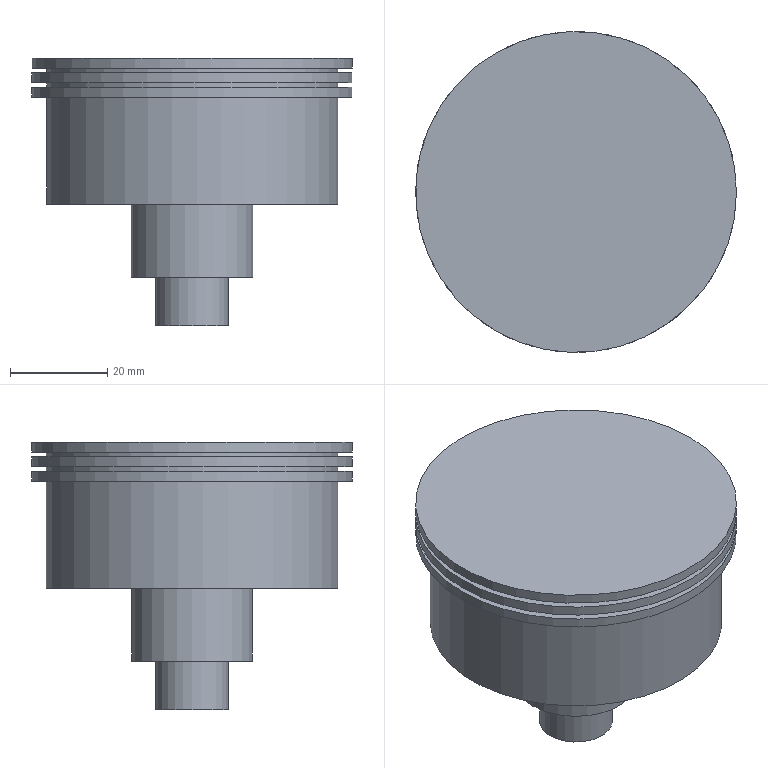Component | NX | AIR_PUMP | 1 solid | 17 faces | box 66 x 66 x 55 mm | volume 97516 mm3 | plane 9 | cylinder 8 | commonest cylinder face diameters 66 x3 60 x3 25 x1 15 x1
STEP:
#1=CARTESIAN_POINT('',(0.,0.,0.));
#2=DIRECTION('',(0.,0.,1.));
#3=DIRECTION('',(1.,0.,0.));
#4=AXIS2_PLACEMENT_3D('',#1,#2,#3);
#5=CARTESIAN_POINT('',(73.907,-56.768,202.5));
#6=VERTEX_POINT('',#5);
#7=CARTESIAN_POINT('',(70.,-24.,202.5));
#8=DIRECTION('',(0.,0.,-1.));
#9=DIRECTION('',(0.1184,-0.993,0.));
#10=AXIS2_PLACEMENT_3D('',#7,#8,#9);
#11=CIRCLE('',#10,33.);
#12=CARTESIAN_POINT('',(70.,-24.,202.5));
#13=DIRECTION('',(0.,0.,1.));
#14=DIRECTION('',(0.1184,-0.993,0.));
#15=AXIS2_PLACEMENT_3D('',#12,#13,#14);
#16=PLANE('',#15);
#17=CARTESIAN_POINT('',(33.,0.));
#18=CARTESIAN_POINT('',(33.,-57.158));
#19=CARTESIAN_POINT('',(-16.5,-28.579));
#20=CARTESIAN_POINT('',(-66.,-0.));
#21=CARTESIAN_POINT('',(-16.5,28.579));
#22=CARTESIAN_POINT('',(33.,57.158));
#23=CARTESIAN_POINT('',(33.,0.));
#24=(BOUNDED_CURVE()B_SPLINE_CURVE(2,(#17,#18,#19,#20,#21,#22,#23),.UNSPECIFIED.,.T.,.F.)B_SPLINE_CURVE_WITH_KNOTS((1,2,2,2,2,1),(-2.094,0.,2.094,4.189,6.283,8.378),.UNSPECIFIED.)CURVE()GEOMETRIC_REPRESENTATION_ITEM()RATIONAL_B_SPLINE_CURVE((1.,0.5,1.,0.5,1.,0.5,1.))REPRESENTATION_ITEM(''));
#25=(GEOMETRIC_REPRESENTATION_CONTEXT(2)PARAMETRIC_REPRESENTATION_CONTEXT()REPRESENTATION_CONTEXT('',''));
#26=DEFINITIONAL_REPRESENTATION('',(#24),#25);
#27=PCURVE('',#16,#26);
#28=CARTESIAN_POINT('',(70.,-24.,200.5));
#29=DIRECTION('',(0.,0.,1.));
#30=DIRECTION('',(0.1184,-0.993,0.));
#31=AXIS2_PLACEMENT_3D('',#28,#29,#30);
#32=CYLINDRICAL_SURFACE('',#31,33.);
#33=CARTESIAN_POINT('',(6.283,2.));
#34=DIRECTION('',(-1.,0.));
#35=VECTOR('',#34,1.);
#36=LINE('',#33,#35);
#37=(GEOMETRIC_REPRESENTATION_CONTEXT(2)PARAMETRIC_REPRESENTATION_CONTEXT()REPRESENTATION_CONTEXT('',''));
#38=DEFINITIONAL_REPRESENTATION('',(#36),#37);
#39=PCURVE('',#32,#38);
#40=SURFACE_CURVE('',#11,(#27,#39),.PCURVE_S1.);
#41=EDGE_CURVE('',#6,#6,#40,.T.);
#42=ORIENTED_EDGE('',*,*,#41,.F.);
#43=EDGE_LOOP('',(#42));
#44=FACE_BOUND('',#43,.T.);
#45=ADVANCED_FACE('',(#44),#16,.T.);
#46=CARTESIAN_POINT('',(66.448,5.789,200.5));
#47=VERTEX_POINT('',#46);
#48=CARTESIAN_POINT('',(70.,-24.,200.5));
#49=DIRECTION('',(0.,0.,-1.));
#50=DIRECTION('',(-0.1184,0.993,0.));
#51=AXIS2_PLACEMENT_3D('',#48,#49,#50);
#52=CIRCLE('',#51,30.);
#53=CARTESIAN_POINT('',(70.,-24.,200.5));
#54=DIRECTION('',(0.,0.,-1.));
#55=DIRECTION('',(-0.1184,0.993,0.));
#56=AXIS2_PLACEMENT_3D('',#53,#54,#55);
#57=PLANE('',#56);
#58=CARTESIAN_POINT('',(0.,0.));
#59=DIRECTION('',(1.,0.));
#60=AXIS2_PLACEMENT_2D('',#58,#59);
#61=CIRCLE('',#60,30.);
#62=(GEOMETRIC_REPRESENTATION_CONTEXT(2)PARAMETRIC_REPRESENTATION_CONTEXT()REPRESENTATION_CONTEXT('',''));
#63=DEFINITIONAL_REPRESENTATION('',(#61),#62);
#64=PCURVE('',#57,#63);
#65=CARTESIAN_POINT('',(70.,-24.,200.5));
#66=DIRECTION('',(0.,0.,-1.));
#67=DIRECTION('',(-0.1184,0.993,0.));
#68=AXIS2_PLACEMENT_3D('',#65,#66,#67);
#69=CYLINDRICAL_SURFACE('',#68,30.);
#70=CARTESIAN_POINT('',(0.,0.));
#71=DIRECTION('',(1.,0.));
#72=VECTOR('',#71,1.);
#73=LINE('',#70,#72);
#74=(GEOMETRIC_REPRESENTATION_CONTEXT(2)PARAMETRIC_REPRESENTATION_CONTEXT()REPRESENTATION_CONTEXT('',''));
#75=DEFINITIONAL_REPRESENTATION('',(#73),#74);
#76=PCURVE('',#69,#75);
#77=SURFACE_CURVE('',#52,(#64,#76),.PCURVE_S1.);
#78=EDGE_CURVE('',#47,#47,#77,.T.);
#79=ORIENTED_EDGE('',*,*,#78,.F.);
#80=EDGE_LOOP('',(#79));
#81=FACE_BOUND('',#80,.T.);
#82=CARTESIAN_POINT('',(73.907,-56.768,200.5));
#83=VERTEX_POINT('',#82);
#84=CARTESIAN_POINT('',(70.,-24.,200.5));
#85=DIRECTION('',(0.,0.,1.));
#86=DIRECTION('',(0.1184,-0.993,0.));
#87=AXIS2_PLACEMENT_3D('',#84,#85,#86);
#88=CIRCLE('',#87,33.);
#89=CARTESIAN_POINT('',(-33.,0.));
#90=CARTESIAN_POINT('',(-33.,57.158));
#91=CARTESIAN_POINT('',(16.5,28.579));
#92=CARTESIAN_POINT('',(66.,0.));
#93=CARTESIAN_POINT('',(16.5,-28.579));
#94=CARTESIAN_POINT('',(-33.,-57.158));
#95=CARTESIAN_POINT('',(-33.,0.));
#96=(BOUNDED_CURVE()B_SPLINE_CURVE(2,(#89,#90,#91,#92,#93,#94,#95),.UNSPECIFIED.,.T.,.F.)B_SPLINE_CURVE_WITH_KNOTS((1,2,2,2,2,1),(-2.094,0.,2.094,4.189,6.283,8.378),.UNSPECIFIED.)CURVE()GEOMETRIC_REPRESENTATION_ITEM()RATIONAL_B_SPLINE_CURVE((1.,0.5,1.,0.5,1.,0.5,1.))REPRESENTATION_ITEM(''));
#97=(GEOMETRIC_REPRESENTATION_CONTEXT(2)PARAMETRIC_REPRESENTATION_CONTEXT()REPRESENTATION_CONTEXT('',''));
#98=DEFINITIONAL_REPRESENTATION('',(#96),#97);
#99=PCURVE('',#57,#98);
#100=CARTESIAN_POINT('',(0.,0.));
#101=DIRECTION('',(1.,0.));
#102=VECTOR('',#101,1.);
#103=LINE('',#100,#102);
#104=(GEOMETRIC_REPRESENTATION_CONTEXT(2)PARAMETRIC_REPRESENTATION_CONTEXT()REPRESENTATION_CONTEXT('',''));
#105=DEFINITIONAL_REPRESENTATION('',(#103),#104);
#106=PCURVE('',#32,#105);
#107=SURFACE_CURVE('',#88,(#99,#106),.PCURVE_S1.);
#108=EDGE_CURVE('',#83,#83,#107,.T.);
#109=ORIENTED_EDGE('',*,*,#108,.F.);
#110=EDGE_LOOP('',(#109));
#111=FACE_BOUND('',#110,.T.);
#112=ADVANCED_FACE('',(#81,#111),#57,.T.);
#113=ORIENTED_EDGE('',*,*,#41,.T.);
#114=CARTESIAN_POINT('',(73.907,-56.768,200.5));
#115=CARTESIAN_POINT('',(73.907,-56.768,202.5));
#116=B_SPLINE_CURVE_WITH_KNOTS('',1,(#114,#115),.UNSPECIFIED.,.F.,.F.,(2,2),(0.,2.),.PIECEWISE_BEZIER_KNOTS.);
#117=CARTESIAN_POINT('',(0.,0.));
#118=DIRECTION('',(0.,1.));
#119=VECTOR('',#118,1.);
#120=LINE('',#117,#119);
#121=(GEOMETRIC_REPRESENTATION_CONTEXT(2)PARAMETRIC_REPRESENTATION_CONTEXT()REPRESENTATION_CONTEXT('',''));
#122=DEFINITIONAL_REPRESENTATION('',(#120),#121);
#123=PCURVE('',#32,#122);
#124=CARTESIAN_POINT('',(6.283,0.));
#125=DIRECTION('',(0.,1.));
#126=VECTOR('',#125,1.);
#127=LINE('',#124,#126);
#128=(GEOMETRIC_REPRESENTATION_CONTEXT(2)PARAMETRIC_REPRESENTATION_CONTEXT()REPRESENTATION_CONTEXT('',''));
#129=DEFINITIONAL_REPRESENTATION('',(#127),#128);
#130=PCURVE('',#32,#129);
#131=SEAM_CURVE('',#116,(#123,#130),.PCURVE_S1.);
#132=EDGE_CURVE('',#83,#6,#131,.T.);
#133=ORIENTED_EDGE('',*,*,#132,.F.);
#134=ORIENTED_EDGE('',*,*,#108,.T.);
#135=ORIENTED_EDGE('',*,*,#132,.T.);
#136=EDGE_LOOP('',(#113,#133,#134,#135));
#137=FACE_BOUND('',#136,.T.);
#138=ADVANCED_FACE('',(#137),#32,.T.);
#139=CARTESIAN_POINT('',(66.448,5.789,199.5));
#140=VERTEX_POINT('',#139);
#141=CARTESIAN_POINT('',(70.,-24.,199.5));
#142=DIRECTION('',(0.,0.,-1.));
#143=DIRECTION('',(-0.1184,0.993,0.));
#144=AXIS2_PLACEMENT_3D('',#141,#142,#143);
#145=CIRCLE('',#144,30.);
#146=CARTESIAN_POINT('',(0.,1.));
#147=DIRECTION('',(1.,0.));
#148=VECTOR('',#147,1.);
#149=LINE('',#146,#148);
#150=(GEOMETRIC_REPRESENTATION_CONTEXT(2)PARAMETRIC_REPRESENTATION_CONTEXT()REPRESENTATION_CONTEXT('',''));
#151=DEFINITIONAL_REPRESENTATION('',(#149),#150);
#152=PCURVE('',#69,#151);
#153=CARTESIAN_POINT('',(70.,-24.,199.5));
#154=DIRECTION('',(0.,0.,1.));
#155=DIRECTION('',(0.1184,-0.993,0.));
#156=AXIS2_PLACEMENT_3D('',#153,#154,#155);
#157=PLANE('',#156);
#158=CARTESIAN_POINT('',(-30.,0.));
#159=CARTESIAN_POINT('',(-30.,51.962));
#160=CARTESIAN_POINT('',(15.,25.981));
#161=CARTESIAN_POINT('',(60.,0.));
#162=CARTESIAN_POINT('',(15.,-25.981));
#163=CARTESIAN_POINT('',(-30.,-51.962));
#164=CARTESIAN_POINT('',(-30.,0.));
#165=(BOUNDED_CURVE()B_SPLINE_CURVE(2,(#158,#159,#160,#161,#162,#163,#164),.UNSPECIFIED.,.T.,.F.)B_SPLINE_CURVE_WITH_KNOTS((1,2,2,2,2,1),(-2.094,0.,2.094,4.189,6.283,8.378),.UNSPECIFIED.)CURVE()GEOMETRIC_REPRESENTATION_ITEM()RATIONAL_B_SPLINE_CURVE((1.,0.5,1.,0.5,1.,0.5,1.))REPRESENTATION_ITEM(''));
#166=(GEOMETRIC_REPRESENTATION_CONTEXT(2)PARAMETRIC_REPRESENTATION_CONTEXT()REPRESENTATION_CONTEXT('',''));
#167=DEFINITIONAL_REPRESENTATION('',(#165),#166);
#168=PCURVE('',#157,#167);
#169=SURFACE_CURVE('',#145,(#152,#168),.PCURVE_S1.);
#170=EDGE_CURVE('',#140,#140,#169,.T.);
#171=ORIENTED_EDGE('',*,*,#170,.F.);
#172=CARTESIAN_POINT('',(66.448,5.789,200.5));
#173=CARTESIAN_POINT('',(66.448,5.789,199.5));
#174=B_SPLINE_CURVE_WITH_KNOTS('',1,(#172,#173),.UNSPECIFIED.,.F.,.F.,(2,2),(0.,1.),.PIECEWISE_BEZIER_KNOTS.);
#175=CARTESIAN_POINT('',(0.,0.));
#176=DIRECTION('',(0.,1.));
#177=VECTOR('',#176,1.);
#178=LINE('',#175,#177);
#179=(GEOMETRIC_REPRESENTATION_CONTEXT(2)PARAMETRIC_REPRESENTATION_CONTEXT()REPRESENTATION_CONTEXT('',''));
#180=DEFINITIONAL_REPRESENTATION('',(#178),#179);
#181=PCURVE('',#69,#180);
#182=CARTESIAN_POINT('',(6.283,0.));
#183=DIRECTION('',(0.,1.));
#184=VECTOR('',#183,1.);
#185=LINE('',#182,#184);
#186=(GEOMETRIC_REPRESENTATION_CONTEXT(2)PARAMETRIC_REPRESENTATION_CONTEXT()REPRESENTATION_CONTEXT('',''));
#187=DEFINITIONAL_REPRESENTATION('',(#185),#186);
#188=PCURVE('',#69,#187);
#189=SEAM_CURVE('',#174,(#181,#188),.PCURVE_S1.);
#190=EDGE_CURVE('',#47,#140,#189,.T.);
#191=ORIENTED_EDGE('',*,*,#190,.F.);
#192=ORIENTED_EDGE('',*,*,#78,.T.);
#193=ORIENTED_EDGE('',*,*,#190,.T.);
#194=EDGE_LOOP('',(#171,#191,#192,#193));
#195=FACE_BOUND('',#194,.T.);
#196=ADVANCED_FACE('',(#195),#69,.T.);
#197=CARTESIAN_POINT('',(66.448,5.789,197.5));
#198=VERTEX_POINT('',#197);
#199=CARTESIAN_POINT('',(70.,-24.,197.5));
#200=DIRECTION('',(0.,0.,-1.));
#201=DIRECTION('',(-0.1184,0.993,0.));
#202=AXIS2_PLACEMENT_3D('',#199,#200,#201);
#203=CIRCLE('',#202,30.);
#204=CARTESIAN_POINT('',(70.,-24.,197.5));
#205=DIRECTION('',(0.,0.,-1.));
#206=DIRECTION('',(-0.1184,0.993,0.));
#207=AXIS2_PLACEMENT_3D('',#204,#205,#206);
#208=PLANE('',#207);
#209=CARTESIAN_POINT('',(0.,0.));
#210=DIRECTION('',(1.,0.));
#211=AXIS2_PLACEMENT_2D('',#209,#210);
#212=CIRCLE('',#211,30.);
#213=(GEOMETRIC_REPRESENTATION_CONTEXT(2)PARAMETRIC_REPRESENTATION_CONTEXT()REPRESENTATION_CONTEXT('',''));
#214=DEFINITIONAL_REPRESENTATION('',(#212),#213);
#215=PCURVE('',#208,#214);
#216=CARTESIAN_POINT('',(70.,-24.,197.5));
#217=DIRECTION('',(0.,0.,-1.));
#218=DIRECTION('',(-0.1184,0.993,0.));
#219=AXIS2_PLACEMENT_3D('',#216,#217,#218);
#220=CYLINDRICAL_SURFACE('',#219,30.);
#221=CARTESIAN_POINT('',(0.,0.));
#222=DIRECTION('',(1.,0.));
#223=VECTOR('',#222,1.);
#224=LINE('',#221,#223);
#225=(GEOMETRIC_REPRESENTATION_CONTEXT(2)PARAMETRIC_REPRESENTATION_CONTEXT()REPRESENTATION_CONTEXT('',''));
#226=DEFINITIONAL_REPRESENTATION('',(#224),#225);
#227=PCURVE('',#220,#226);
#228=SURFACE_CURVE('',#203,(#215,#227),.PCURVE_S1.);
#229=EDGE_CURVE('',#198,#198,#228,.T.);
#230=ORIENTED_EDGE('',*,*,#229,.F.);
#231=EDGE_LOOP('',(#230));
#232=FACE_BOUND('',#231,.T.);
#233=CARTESIAN_POINT('',(66.093,8.768,197.5));
#234=VERTEX_POINT('',#233);
#235=CARTESIAN_POINT('',(70.,-24.,197.5));
#236=DIRECTION('',(0.,0.,-1.));
#237=DIRECTION('',(-0.1184,0.993,0.));
#238=AXIS2_PLACEMENT_3D('',#235,#236,#237);
#239=CIRCLE('',#238,33.);
#240=CARTESIAN_POINT('',(0.,0.));
#241=DIRECTION('',(1.,0.));
#242=AXIS2_PLACEMENT_2D('',#240,#241);
#243=CIRCLE('',#242,33.);
#244=(GEOMETRIC_REPRESENTATION_CONTEXT(2)PARAMETRIC_REPRESENTATION_CONTEXT()REPRESENTATION_CONTEXT('',''));
#245=DEFINITIONAL_REPRESENTATION('',(#243),#244);
#246=PCURVE('',#208,#245);
#247=CARTESIAN_POINT('',(70.,-24.,199.5));
#248=DIRECTION('',(0.,0.,-1.));
#249=DIRECTION('',(-0.1184,0.993,0.));
#250=AXIS2_PLACEMENT_3D('',#247,#248,#249);
#251=CYLINDRICAL_SURFACE('',#250,33.);
#252=CARTESIAN_POINT('',(0.,2.));
#253=DIRECTION('',(1.,0.));
#254=VECTOR('',#253,1.);
#255=LINE('',#252,#254);
#256=(GEOMETRIC_REPRESENTATION_CONTEXT(2)PARAMETRIC_REPRESENTATION_CONTEXT()REPRESENTATION_CONTEXT('',''));
#257=DEFINITIONAL_REPRESENTATION('',(#255),#256);
#258=PCURVE('',#251,#257);
#259=SURFACE_CURVE('',#239,(#246,#258),.PCURVE_S1.);
#260=EDGE_CURVE('',#234,#234,#259,.T.);
#261=ORIENTED_EDGE('',*,*,#260,.T.);
#262=EDGE_LOOP('',(#261));
#263=FACE_BOUND('',#262,.T.);
#264=ADVANCED_FACE('',(#232,#263),#208,.T.);
#265=ORIENTED_EDGE('',*,*,#170,.T.);
#266=EDGE_LOOP('',(#265));
#267=FACE_BOUND('',#266,.T.);
#268=CARTESIAN_POINT('',(66.093,8.768,199.5));
#269=VERTEX_POINT('',#268);
#270=CARTESIAN_POINT('',(70.,-24.,199.5));
#271=DIRECTION('',(0.,0.,-1.));
#272=DIRECTION('',(-0.1184,0.993,0.));
#273=AXIS2_PLACEMENT_3D('',#270,#271,#272);
#274=CIRCLE('',#273,33.);
#275=CARTESIAN_POINT('',(-33.,0.));
#276=CARTESIAN_POINT('',(-33.,57.158));
#277=CARTESIAN_POINT('',(16.5,28.579));
#278=CARTESIAN_POINT('',(66.,0.));
#279=CARTESIAN_POINT('',(16.5,-28.579));
#280=CARTESIAN_POINT('',(-33.,-57.158));
#281=CARTESIAN_POINT('',(-33.,0.));
#282=(BOUNDED_CURVE()B_SPLINE_CURVE(2,(#275,#276,#277,#278,#279,#280,#281),.UNSPECIFIED.,.T.,.F.)B_SPLINE_CURVE_WITH_KNOTS((1,2,2,2,2,1),(-2.094,0.,2.094,4.189,6.283,8.378),.UNSPECIFIED.)CURVE()GEOMETRIC_REPRESENTATION_ITEM()RATIONAL_B_SPLINE_CURVE((1.,0.5,1.,0.5,1.,0.5,1.))REPRESENTATION_ITEM(''));
#283=(GEOMETRIC_REPRESENTATION_CONTEXT(2)PARAMETRIC_REPRESENTATION_CONTEXT()REPRESENTATION_CONTEXT('',''));
#284=DEFINITIONAL_REPRESENTATION('',(#282),#283);
#285=PCURVE('',#157,#284);
#286=CARTESIAN_POINT('',(0.,0.));
#287=DIRECTION('',(1.,0.));
#288=VECTOR('',#287,1.);
#289=LINE('',#286,#288);
#290=(GEOMETRIC_REPRESENTATION_CONTEXT(2)PARAMETRIC_REPRESENTATION_CONTEXT()REPRESENTATION_CONTEXT('',''));
#291=DEFINITIONAL_REPRESENTATION('',(#289),#290);
#292=PCURVE('',#251,#291);
#293=SURFACE_CURVE('',#274,(#285,#292),.PCURVE_S1.);
#294=EDGE_CURVE('',#269,#269,#293,.T.);
#295=ORIENTED_EDGE('',*,*,#294,.F.);
#296=EDGE_LOOP('',(#295));
#297=FACE_BOUND('',#296,.T.);
#298=ADVANCED_FACE('',(#267,#297),#157,.T.);
#299=ORIENTED_EDGE('',*,*,#260,.F.);
#300=CARTESIAN_POINT('',(66.093,8.768,199.5));
#301=CARTESIAN_POINT('',(66.093,8.768,197.5));
#302=B_SPLINE_CURVE_WITH_KNOTS('',1,(#300,#301),.UNSPECIFIED.,.F.,.F.,(2,2),(0.,2.),.PIECEWISE_BEZIER_KNOTS.);
#303=CARTESIAN_POINT('',(0.,0.));
#304=DIRECTION('',(0.,1.));
#305=VECTOR('',#304,1.);
#306=LINE('',#303,#305);
#307=(GEOMETRIC_REPRESENTATION_CONTEXT(2)PARAMETRIC_REPRESENTATION_CONTEXT()REPRESENTATION_CONTEXT('',''));
#308=DEFINITIONAL_REPRESENTATION('',(#306),#307);
#309=PCURVE('',#251,#308);
#310=CARTESIAN_POINT('',(6.283,0.));
#311=DIRECTION('',(0.,1.));
#312=VECTOR('',#311,1.);
#313=LINE('',#310,#312);
#314=(GEOMETRIC_REPRESENTATION_CONTEXT(2)PARAMETRIC_REPRESENTATION_CONTEXT()REPRESENTATION_CONTEXT('',''));
#315=DEFINITIONAL_REPRESENTATION('',(#313),#314);
#316=PCURVE('',#251,#315);
#317=SEAM_CURVE('',#302,(#309,#316),.PCURVE_S1.);
#318=EDGE_CURVE('',#269,#234,#317,.T.);
#319=ORIENTED_EDGE('',*,*,#318,.F.);
#320=ORIENTED_EDGE('',*,*,#294,.T.);
#321=ORIENTED_EDGE('',*,*,#318,.T.);
#322=EDGE_LOOP('',(#299,#319,#320,#321));
#323=FACE_BOUND('',#322,.T.);
#324=ADVANCED_FACE('',(#323),#251,.T.);
#325=CARTESIAN_POINT('',(66.448,5.789,196.5));
#326=VERTEX_POINT('',#325);
#327=CARTESIAN_POINT('',(70.,-24.,196.5));
#328=DIRECTION('',(0.,0.,-1.));
#329=DIRECTION('',(-0.1184,0.993,0.));
#330=AXIS2_PLACEMENT_3D('',#327,#328,#329);
#331=CIRCLE('',#330,30.);
#332=CARTESIAN_POINT('',(0.,1.));
#333=DIRECTION('',(1.,0.));
#334=VECTOR('',#333,1.);
#335=LINE('',#332,#334);
#336=(GEOMETRIC_REPRESENTATION_CONTEXT(2)PARAMETRIC_REPRESENTATION_CONTEXT()REPRESENTATION_CONTEXT('',''));
#337=DEFINITIONAL_REPRESENTATION('',(#335),#336);
#338=PCURVE('',#220,#337);
#339=CARTESIAN_POINT('',(70.,-24.,196.5));
#340=DIRECTION('',(0.,0.,1.));
#341=DIRECTION('',(0.1184,-0.993,0.));
#342=AXIS2_PLACEMENT_3D('',#339,#340,#341);
#343=PLANE('',#342);
#344=CARTESIAN_POINT('',(-30.,0.));
#345=CARTESIAN_POINT('',(-30.,51.962));
#346=CARTESIAN_POINT('',(15.,25.981));
#347=CARTESIAN_POINT('',(60.,0.));
#348=CARTESIAN_POINT('',(15.,-25.981));
#349=CARTESIAN_POINT('',(-30.,-51.962));
#350=CARTESIAN_POINT('',(-30.,0.));
#351=(BOUNDED_CURVE()B_SPLINE_CURVE(2,(#344,#345,#346,#347,#348,#349,#350),.UNSPECIFIED.,.T.,.F.)B_SPLINE_CURVE_WITH_KNOTS((1,2,2,2,2,1),(-2.094,0.,2.094,4.189,6.283,8.378),.UNSPECIFIED.)CURVE()GEOMETRIC_REPRESENTATION_ITEM()RATIONAL_B_SPLINE_CURVE((1.,0.5,1.,0.5,1.,0.5,1.))REPRESENTATION_ITEM(''));
#352=(GEOMETRIC_REPRESENTATION_CONTEXT(2)PARAMETRIC_REPRESENTATION_CONTEXT()REPRESENTATION_CONTEXT('',''));
#353=DEFINITIONAL_REPRESENTATION('',(#351),#352);
#354=PCURVE('',#343,#353);
#355=SURFACE_CURVE('',#331,(#338,#354),.PCURVE_S1.);
#356=EDGE_CURVE('',#326,#326,#355,.T.);
#357=ORIENTED_EDGE('',*,*,#356,.F.);
#358=CARTESIAN_POINT('',(66.448,5.789,197.5));
#359=CARTESIAN_POINT('',(66.448,5.789,196.5));
#360=B_SPLINE_CURVE_WITH_KNOTS('',1,(#358,#359),.UNSPECIFIED.,.F.,.F.,(2,2),(0.,1.),.PIECEWISE_BEZIER_KNOTS.);
#361=CARTESIAN_POINT('',(0.,0.));
#362=DIRECTION('',(0.,1.));
#363=VECTOR('',#362,1.);
#364=LINE('',#361,#363);
#365=(GEOMETRIC_REPRESENTATION_CONTEXT(2)PARAMETRIC_REPRESENTATION_CONTEXT()REPRESENTATION_CONTEXT('',''));
#366=DEFINITIONAL_REPRESENTATION('',(#364),#365);
#367=PCURVE('',#220,#366);
#368=CARTESIAN_POINT('',(6.283,0.));
#369=DIRECTION('',(0.,1.));
#370=VECTOR('',#369,1.);
#371=LINE('',#368,#370);
#372=(GEOMETRIC_REPRESENTATION_CONTEXT(2)PARAMETRIC_REPRESENTATION_CONTEXT()REPRESENTATION_CONTEXT('',''));
#373=DEFINITIONAL_REPRESENTATION('',(#371),#372);
#374=PCURVE('',#220,#373);
#375=SEAM_CURVE('',#360,(#367,#374),.PCURVE_S1.);
#376=EDGE_CURVE('',#198,#326,#375,.T.);
#377=ORIENTED_EDGE('',*,*,#376,.F.);
#378=ORIENTED_EDGE('',*,*,#229,.T.);
#379=ORIENTED_EDGE('',*,*,#376,.T.);
#380=EDGE_LOOP('',(#357,#377,#378,#379));
#381=FACE_BOUND('',#380,.T.);
#382=ADVANCED_FACE('',(#381),#220,.T.);
#383=CARTESIAN_POINT('',(66.448,5.789,194.5));
#384=VERTEX_POINT('',#383);
#385=CARTESIAN_POINT('',(70.,-24.,194.5));
#386=DIRECTION('',(0.,0.,-1.));
#387=DIRECTION('',(-0.1184,0.993,0.));
#388=AXIS2_PLACEMENT_3D('',#385,#386,#387);
#389=CIRCLE('',#388,30.);
#390=CARTESIAN_POINT('',(70.,-24.,194.5));
#391=DIRECTION('',(0.,0.,-1.));
#392=DIRECTION('',(-0.1184,0.993,0.));
#393=AXIS2_PLACEMENT_3D('',#390,#391,#392);
#394=PLANE('',#393);
#395=CARTESIAN_POINT('',(0.,0.));
#396=DIRECTION('',(1.,0.));
#397=AXIS2_PLACEMENT_2D('',#395,#396);
#398=CIRCLE('',#397,30.);
#399=(GEOMETRIC_REPRESENTATION_CONTEXT(2)PARAMETRIC_REPRESENTATION_CONTEXT()REPRESENTATION_CONTEXT('',''));
#400=DEFINITIONAL_REPRESENTATION('',(#398),#399);
#401=PCURVE('',#394,#400);
#402=CARTESIAN_POINT('',(70.,-24.,194.5));
#403=DIRECTION('',(0.,0.,-1.));
#404=DIRECTION('',(-0.1184,0.993,0.));
#405=AXIS2_PLACEMENT_3D('',#402,#403,#404);
#406=CYLINDRICAL_SURFACE('',#405,30.);
#407=CARTESIAN_POINT('',(0.,0.));
#408=DIRECTION('',(1.,0.));
#409=VECTOR('',#408,1.);
#410=LINE('',#407,#409);
#411=(GEOMETRIC_REPRESENTATION_CONTEXT(2)PARAMETRIC_REPRESENTATION_CONTEXT()REPRESENTATION_CONTEXT('',''));
#412=DEFINITIONAL_REPRESENTATION('',(#410),#411);
#413=PCURVE('',#406,#412);
#414=SURFACE_CURVE('',#389,(#401,#413),.PCURVE_S1.);
#415=EDGE_CURVE('',#384,#384,#414,.T.);
#416=ORIENTED_EDGE('',*,*,#415,.F.);
#417=EDGE_LOOP('',(#416));
#418=FACE_BOUND('',#417,.T.);
#419=CARTESIAN_POINT('',(66.093,8.768,194.5));
#420=VERTEX_POINT('',#419);
#421=CARTESIAN_POINT('',(70.,-24.,194.5));
#422=DIRECTION('',(0.,0.,-1.));
#423=DIRECTION('',(-0.1184,0.993,0.));
#424=AXIS2_PLACEMENT_3D('',#421,#422,#423);
#425=CIRCLE('',#424,33.);
#426=CARTESIAN_POINT('',(0.,0.));
#427=DIRECTION('',(1.,0.));
#428=AXIS2_PLACEMENT_2D('',#426,#427);
#429=CIRCLE('',#428,33.);
#430=(GEOMETRIC_REPRESENTATION_CONTEXT(2)PARAMETRIC_REPRESENTATION_CONTEXT()REPRESENTATION_CONTEXT('',''));
#431=DEFINITIONAL_REPRESENTATION('',(#429),#430);
#432=PCURVE('',#394,#431);
#433=CARTESIAN_POINT('',(70.,-24.,196.5));
#434=DIRECTION('',(0.,0.,-1.));
#435=DIRECTION('',(-0.1184,0.993,0.));
#436=AXIS2_PLACEMENT_3D('',#433,#434,#435);
#437=CYLINDRICAL_SURFACE('',#436,33.);
#438=CARTESIAN_POINT('',(0.,2.));
#439=DIRECTION('',(1.,0.));
#440=VECTOR('',#439,1.);
#441=LINE('',#438,#440);
#442=(GEOMETRIC_REPRESENTATION_CONTEXT(2)PARAMETRIC_REPRESENTATION_CONTEXT()REPRESENTATION_CONTEXT('',''));
#443=DEFINITIONAL_REPRESENTATION('',(#441),#442);
#444=PCURVE('',#437,#443);
#445=SURFACE_CURVE('',#425,(#432,#444),.PCURVE_S1.);
#446=EDGE_CURVE('',#420,#420,#445,.T.);
#447=ORIENTED_EDGE('',*,*,#446,.T.);
#448=EDGE_LOOP('',(#447));
#449=FACE_BOUND('',#448,.T.);
#450=ADVANCED_FACE('',(#418,#449),#394,.T.);
#451=ORIENTED_EDGE('',*,*,#356,.T.);
#452=EDGE_LOOP('',(#451));
#453=FACE_BOUND('',#452,.T.);
#454=CARTESIAN_POINT('',(66.093,8.768,196.5));
#455=VERTEX_POINT('',#454);
#456=CARTESIAN_POINT('',(70.,-24.,196.5));
#457=DIRECTION('',(0.,0.,-1.));
#458=DIRECTION('',(-0.1184,0.993,0.));
#459=AXIS2_PLACEMENT_3D('',#456,#457,#458);
#460=CIRCLE('',#459,33.);
#461=CARTESIAN_POINT('',(-33.,0.));
#462=CARTESIAN_POINT('',(-33.,57.158));
#463=CARTESIAN_POINT('',(16.5,28.579));
#464=CARTESIAN_POINT('',(66.,0.));
#465=CARTESIAN_POINT('',(16.5,-28.579));
#466=CARTESIAN_POINT('',(-33.,-57.158));
#467=CARTESIAN_POINT('',(-33.,0.));
#468=(BOUNDED_CURVE()B_SPLINE_CURVE(2,(#461,#462,#463,#464,#465,#466,#467),.UNSPECIFIED.,.T.,.F.)B_SPLINE_CURVE_WITH_KNOTS((1,2,2,2,2,1),(-2.094,0.,2.094,4.189,6.283,8.378),.UNSPECIFIED.)CURVE()GEOMETRIC_REPRESENTATION_ITEM()RATIONAL_B_SPLINE_CURVE((1.,0.5,1.,0.5,1.,0.5,1.))REPRESENTATION_ITEM(''));
#469=(GEOMETRIC_REPRESENTATION_CONTEXT(2)PARAMETRIC_REPRESENTATION_CONTEXT()REPRESENTATION_CONTEXT('',''));
#470=DEFINITIONAL_REPRESENTATION('',(#468),#469);
#471=PCURVE('',#343,#470);
#472=CARTESIAN_POINT('',(0.,0.));
#473=DIRECTION('',(1.,0.));
#474=VECTOR('',#473,1.);
#475=LINE('',#472,#474);
#476=(GEOMETRIC_REPRESENTATION_CONTEXT(2)PARAMETRIC_REPRESENTATION_CONTEXT()REPRESENTATION_CONTEXT('',''));
#477=DEFINITIONAL_REPRESENTATION('',(#475),#476);
#478=PCURVE('',#437,#477);
#479=SURFACE_CURVE('',#460,(#471,#478),.PCURVE_S1.);
#480=EDGE_CURVE('',#455,#455,#479,.T.);
#481=ORIENTED_EDGE('',*,*,#480,.F.);
#482=EDGE_LOOP('',(#481));
#483=FACE_BOUND('',#482,.T.);
#484=ADVANCED_FACE('',(#453,#483),#343,.T.);
#485=ORIENTED_EDGE('',*,*,#446,.F.);
#486=CARTESIAN_POINT('',(66.093,8.768,196.5));
#487=CARTESIAN_POINT('',(66.093,8.768,194.5));
#488=B_SPLINE_CURVE_WITH_KNOTS('',1,(#486,#487),.UNSPECIFIED.,.F.,.F.,(2,2),(0.,2.),.PIECEWISE_BEZIER_KNOTS.);
#489=CARTESIAN_POINT('',(0.,0.));
#490=DIRECTION('',(0.,1.));
#491=VECTOR('',#490,1.);
#492=LINE('',#489,#491);
#493=(GEOMETRIC_REPRESENTATION_CONTEXT(2)PARAMETRIC_REPRESENTATION_CONTEXT()REPRESENTATION_CONTEXT('',''));
#494=DEFINITIONAL_REPRESENTATION('',(#492),#493);
#495=PCURVE('',#437,#494);
#496=CARTESIAN_POINT('',(6.283,0.));
#497=DIRECTION('',(0.,1.));
#498=VECTOR('',#497,1.);
#499=LINE('',#496,#498);
#500=(GEOMETRIC_REPRESENTATION_CONTEXT(2)PARAMETRIC_REPRESENTATION_CONTEXT()REPRESENTATION_CONTEXT('',''));
#501=DEFINITIONAL_REPRESENTATION('',(#499),#500);
#502=PCURVE('',#437,#501);
#503=SEAM_CURVE('',#488,(#495,#502),.PCURVE_S1.);
#504=EDGE_CURVE('',#455,#420,#503,.T.);
#505=ORIENTED_EDGE('',*,*,#504,.F.);
#506=ORIENTED_EDGE('',*,*,#480,.T.);
#507=ORIENTED_EDGE('',*,*,#504,.T.);
#508=EDGE_LOOP('',(#485,#505,#506,#507));
#509=FACE_BOUND('',#508,.T.);
#510=ADVANCED_FACE('',(#509),#437,.T.);
#511=CARTESIAN_POINT('',(68.52,-11.588,172.5));
#512=VERTEX_POINT('',#511);
#513=CARTESIAN_POINT('',(70.,-24.,172.5));
#514=DIRECTION('',(0.,0.,-1.));
#515=DIRECTION('',(-0.1184,0.993,0.));
#516=AXIS2_PLACEMENT_3D('',#513,#514,#515);
#517=CIRCLE('',#516,12.5);
#518=CARTESIAN_POINT('',(70.,-24.,172.5));
#519=DIRECTION('',(0.,0.,-1.));
#520=DIRECTION('',(-0.1184,0.993,0.));
#521=AXIS2_PLACEMENT_3D('',#518,#519,#520);
#522=PLANE('',#521);
#523=CARTESIAN_POINT('',(0.,0.));
#524=DIRECTION('',(1.,0.));
#525=AXIS2_PLACEMENT_2D('',#523,#524);
#526=CIRCLE('',#525,12.5);
#527=(GEOMETRIC_REPRESENTATION_CONTEXT(2)PARAMETRIC_REPRESENTATION_CONTEXT()REPRESENTATION_CONTEXT('',''));
#528=DEFINITIONAL_REPRESENTATION('',(#526),#527);
#529=PCURVE('',#522,#528);
#530=CARTESIAN_POINT('',(70.,-24.,172.5));
#531=DIRECTION('',(0.,0.,-1.));
#532=DIRECTION('',(-0.1184,0.993,0.));
#533=AXIS2_PLACEMENT_3D('',#530,#531,#532);
#534=CYLINDRICAL_SURFACE('',#533,12.5);
#535=CARTESIAN_POINT('',(0.,0.));
#536=DIRECTION('',(1.,0.));
#537=VECTOR('',#536,1.);
#538=LINE('',#535,#537);
#539=(GEOMETRIC_REPRESENTATION_CONTEXT(2)PARAMETRIC_REPRESENTATION_CONTEXT()REPRESENTATION_CONTEXT('',''));
#540=DEFINITIONAL_REPRESENTATION('',(#538),#539);
#541=PCURVE('',#534,#540);
#542=SURFACE_CURVE('',#517,(#529,#541),.PCURVE_S1.);
#543=EDGE_CURVE('',#512,#512,#542,.T.);
#544=ORIENTED_EDGE('',*,*,#543,.F.);
#545=EDGE_LOOP('',(#544));
#546=FACE_BOUND('',#545,.T.);
#547=CARTESIAN_POINT('',(66.448,5.789,172.5));
#548=VERTEX_POINT('',#547);
#549=CARTESIAN_POINT('',(70.,-24.,172.5));
#550=DIRECTION('',(0.,0.,-1.));
#551=DIRECTION('',(-0.1184,0.993,0.));
#552=AXIS2_PLACEMENT_3D('',#549,#550,#551);
#553=CIRCLE('',#552,30.);
#554=CARTESIAN_POINT('',(0.,0.));
#555=DIRECTION('',(1.,0.));
#556=AXIS2_PLACEMENT_2D('',#554,#555);
#557=CIRCLE('',#556,30.);
#558=(GEOMETRIC_REPRESENTATION_CONTEXT(2)PARAMETRIC_REPRESENTATION_CONTEXT()REPRESENTATION_CONTEXT('',''));
#559=DEFINITIONAL_REPRESENTATION('',(#557),#558);
#560=PCURVE('',#522,#559);
#561=CARTESIAN_POINT('',(0.,22.));
#562=DIRECTION('',(1.,0.));
#563=VECTOR('',#562,1.);
#564=LINE('',#561,#563);
#565=(GEOMETRIC_REPRESENTATION_CONTEXT(2)PARAMETRIC_REPRESENTATION_CONTEXT()REPRESENTATION_CONTEXT('',''));
#566=DEFINITIONAL_REPRESENTATION('',(#564),#565);
#567=PCURVE('',#406,#566);
#568=SURFACE_CURVE('',#553,(#560,#567),.PCURVE_S1.);
#569=EDGE_CURVE('',#548,#548,#568,.T.);
#570=ORIENTED_EDGE('',*,*,#569,.T.);
#571=EDGE_LOOP('',(#570));
#572=FACE_BOUND('',#571,.T.);
#573=ADVANCED_FACE('',(#546,#572),#522,.T.);
#574=ORIENTED_EDGE('',*,*,#569,.F.);
#575=CARTESIAN_POINT('',(66.448,5.789,194.5));
#576=CARTESIAN_POINT('',(66.448,5.789,172.5));
#577=B_SPLINE_CURVE_WITH_KNOTS('',1,(#575,#576),.UNSPECIFIED.,.F.,.F.,(2,2),(0.,22.),.PIECEWISE_BEZIER_KNOTS.);
#578=CARTESIAN_POINT('',(0.,0.));
#579=DIRECTION('',(0.,1.));
#580=VECTOR('',#579,1.);
#581=LINE('',#578,#580);
#582=(GEOMETRIC_REPRESENTATION_CONTEXT(2)PARAMETRIC_REPRESENTATION_CONTEXT()REPRESENTATION_CONTEXT('',''));
#583=DEFINITIONAL_REPRESENTATION('',(#581),#582);
#584=PCURVE('',#406,#583);
#585=CARTESIAN_POINT('',(6.283,0.));
#586=DIRECTION('',(0.,1.));
#587=VECTOR('',#586,1.);
#588=LINE('',#585,#587);
#589=(GEOMETRIC_REPRESENTATION_CONTEXT(2)PARAMETRIC_REPRESENTATION_CONTEXT()REPRESENTATION_CONTEXT('',''));
#590=DEFINITIONAL_REPRESENTATION('',(#588),#589);
#591=PCURVE('',#406,#590);
#592=SEAM_CURVE('',#577,(#584,#591),.PCURVE_S1.);
#593=EDGE_CURVE('',#384,#548,#592,.T.);
#594=ORIENTED_EDGE('',*,*,#593,.F.);
#595=ORIENTED_EDGE('',*,*,#415,.T.);
#596=ORIENTED_EDGE('',*,*,#593,.T.);
#597=EDGE_LOOP('',(#574,#594,#595,#596));
#598=FACE_BOUND('',#597,.T.);
#599=ADVANCED_FACE('',(#598),#406,.T.);
#600=CARTESIAN_POINT('',(69.112,-16.553,157.5));
#601=VERTEX_POINT('',#600);
#602=CARTESIAN_POINT('',(70.,-24.,157.5));
#603=DIRECTION('',(0.,0.,-1.));
#604=DIRECTION('',(-0.1184,0.993,0.));
#605=AXIS2_PLACEMENT_3D('',#602,#603,#604);
#606=CIRCLE('',#605,7.5);
#607=CARTESIAN_POINT('',(70.,-24.,157.5));
#608=DIRECTION('',(0.,0.,-1.));
#609=DIRECTION('',(-0.1184,0.993,0.));
#610=AXIS2_PLACEMENT_3D('',#607,#608,#609);
#611=PLANE('',#610);
#612=CARTESIAN_POINT('',(0.,0.));
#613=DIRECTION('',(1.,0.));
#614=AXIS2_PLACEMENT_2D('',#612,#613);
#615=CIRCLE('',#614,7.5);
#616=(GEOMETRIC_REPRESENTATION_CONTEXT(2)PARAMETRIC_REPRESENTATION_CONTEXT()REPRESENTATION_CONTEXT('',''));
#617=DEFINITIONAL_REPRESENTATION('',(#615),#616);
#618=PCURVE('',#611,#617);
#619=CARTESIAN_POINT('',(70.,-24.,157.5));
#620=DIRECTION('',(0.,0.,-1.));
#621=DIRECTION('',(-0.1184,0.993,0.));
#622=AXIS2_PLACEMENT_3D('',#619,#620,#621);
#623=CYLINDRICAL_SURFACE('',#622,7.5);
#624=CARTESIAN_POINT('',(0.,0.));
#625=DIRECTION('',(1.,0.));
#626=VECTOR('',#625,1.);
#627=LINE('',#624,#626);
#628=(GEOMETRIC_REPRESENTATION_CONTEXT(2)PARAMETRIC_REPRESENTATION_CONTEXT()REPRESENTATION_CONTEXT('',''));
#629=DEFINITIONAL_REPRESENTATION('',(#627),#628);
#630=PCURVE('',#623,#629);
#631=SURFACE_CURVE('',#606,(#618,#630),.PCURVE_S1.);
#632=EDGE_CURVE('',#601,#601,#631,.T.);
#633=ORIENTED_EDGE('',*,*,#632,.F.);
#634=EDGE_LOOP('',(#633));
#635=FACE_BOUND('',#634,.T.);
#636=CARTESIAN_POINT('',(68.52,-11.588,157.5));
#637=VERTEX_POINT('',#636);
#638=CARTESIAN_POINT('',(70.,-24.,157.5));
#639=DIRECTION('',(0.,0.,-1.));
#640=DIRECTION('',(-0.1184,0.993,0.));
#641=AXIS2_PLACEMENT_3D('',#638,#639,#640);
#642=CIRCLE('',#641,12.5);
#643=CARTESIAN_POINT('',(0.,0.));
#644=DIRECTION('',(1.,0.));
#645=AXIS2_PLACEMENT_2D('',#643,#644);
#646=CIRCLE('',#645,12.5);
#647=(GEOMETRIC_REPRESENTATION_CONTEXT(2)PARAMETRIC_REPRESENTATION_CONTEXT()REPRESENTATION_CONTEXT('',''));
#648=DEFINITIONAL_REPRESENTATION('',(#646),#647);
#649=PCURVE('',#611,#648);
#650=CARTESIAN_POINT('',(0.,15.));
#651=DIRECTION('',(1.,0.));
#652=VECTOR('',#651,1.);
#653=LINE('',#650,#652);
#654=(GEOMETRIC_REPRESENTATION_CONTEXT(2)PARAMETRIC_REPRESENTATION_CONTEXT()REPRESENTATION_CONTEXT('',''));
#655=DEFINITIONAL_REPRESENTATION('',(#653),#654);
#656=PCURVE('',#534,#655);
#657=SURFACE_CURVE('',#642,(#649,#656),.PCURVE_S1.);
#658=EDGE_CURVE('',#637,#637,#657,.T.);
#659=ORIENTED_EDGE('',*,*,#658,.T.);
#660=EDGE_LOOP('',(#659));
#661=FACE_BOUND('',#660,.T.);
#662=ADVANCED_FACE('',(#635,#661),#611,.T.);
#663=ORIENTED_EDGE('',*,*,#658,.F.);
#664=CARTESIAN_POINT('',(68.52,-11.588,172.5));
#665=CARTESIAN_POINT('',(68.52,-11.588,157.5));
#666=B_SPLINE_CURVE_WITH_KNOTS('',1,(#664,#665),.UNSPECIFIED.,.F.,.F.,(2,2),(0.,15.),.PIECEWISE_BEZIER_KNOTS.);
#667=CARTESIAN_POINT('',(0.,0.));
#668=DIRECTION('',(0.,1.));
#669=VECTOR('',#668,1.);
#670=LINE('',#667,#669);
#671=(GEOMETRIC_REPRESENTATION_CONTEXT(2)PARAMETRIC_REPRESENTATION_CONTEXT()REPRESENTATION_CONTEXT('',''));
#672=DEFINITIONAL_REPRESENTATION('',(#670),#671);
#673=PCURVE('',#534,#672);
#674=CARTESIAN_POINT('',(6.283,0.));
#675=DIRECTION('',(0.,1.));
#676=VECTOR('',#675,1.);
#677=LINE('',#674,#676);
#678=(GEOMETRIC_REPRESENTATION_CONTEXT(2)PARAMETRIC_REPRESENTATION_CONTEXT()REPRESENTATION_CONTEXT('',''));
#679=DEFINITIONAL_REPRESENTATION('',(#677),#678);
#680=PCURVE('',#534,#679);
#681=SEAM_CURVE('',#666,(#673,#680),.PCURVE_S1.);
#682=EDGE_CURVE('',#512,#637,#681,.T.);
#683=ORIENTED_EDGE('',*,*,#682,.F.);
#684=ORIENTED_EDGE('',*,*,#543,.T.);
#685=ORIENTED_EDGE('',*,*,#682,.T.);
#686=EDGE_LOOP('',(#663,#683,#684,#685));
#687=FACE_BOUND('',#686,.T.);
#688=ADVANCED_FACE('',(#687),#534,.T.);
#689=CARTESIAN_POINT('',(69.112,-16.553,147.5));
#690=VERTEX_POINT('',#689);
#691=CARTESIAN_POINT('',(70.,-24.,147.5));
#692=DIRECTION('',(0.,0.,-1.));
#693=DIRECTION('',(-0.1184,0.993,0.));
#694=AXIS2_PLACEMENT_3D('',#691,#692,#693);
#695=CIRCLE('',#694,7.5);
#696=CARTESIAN_POINT('',(70.,-24.,147.5));
#697=DIRECTION('',(0.,0.,-1.));
#698=DIRECTION('',(-0.1184,0.993,0.));
#699=AXIS2_PLACEMENT_3D('',#696,#697,#698);
#700=PLANE('',#699);
#701=CARTESIAN_POINT('',(0.,0.));
#702=DIRECTION('',(1.,0.));
#703=AXIS2_PLACEMENT_2D('',#701,#702);
#704=CIRCLE('',#703,7.5);
#705=(GEOMETRIC_REPRESENTATION_CONTEXT(2)PARAMETRIC_REPRESENTATION_CONTEXT()REPRESENTATION_CONTEXT('',''));
#706=DEFINITIONAL_REPRESENTATION('',(#704),#705);
#707=PCURVE('',#700,#706);
#708=CARTESIAN_POINT('',(0.,10.));
#709=DIRECTION('',(1.,0.));
#710=VECTOR('',#709,1.);
#711=LINE('',#708,#710);
#712=(GEOMETRIC_REPRESENTATION_CONTEXT(2)PARAMETRIC_REPRESENTATION_CONTEXT()REPRESENTATION_CONTEXT('',''));
#713=DEFINITIONAL_REPRESENTATION('',(#711),#712);
#714=PCURVE('',#623,#713);
#715=SURFACE_CURVE('',#695,(#707,#714),.PCURVE_S1.);
#716=EDGE_CURVE('',#690,#690,#715,.T.);
#717=ORIENTED_EDGE('',*,*,#716,.T.);
#718=EDGE_LOOP('',(#717));
#719=FACE_BOUND('',#718,.T.);
#720=ADVANCED_FACE('',(#719),#700,.T.);
#721=ORIENTED_EDGE('',*,*,#716,.F.);
#722=CARTESIAN_POINT('',(69.112,-16.553,157.5));
#723=CARTESIAN_POINT('',(69.112,-16.553,147.5));
#724=B_SPLINE_CURVE_WITH_KNOTS('',1,(#722,#723),.UNSPECIFIED.,.F.,.F.,(2,2),(0.,10.),.PIECEWISE_BEZIER_KNOTS.);
#725=CARTESIAN_POINT('',(0.,0.));
#726=DIRECTION('',(0.,1.));
#727=VECTOR('',#726,1.);
#728=LINE('',#725,#727);
#729=(GEOMETRIC_REPRESENTATION_CONTEXT(2)PARAMETRIC_REPRESENTATION_CONTEXT()REPRESENTATION_CONTEXT('',''));
#730=DEFINITIONAL_REPRESENTATION('',(#728),#729);
#731=PCURVE('',#623,#730);
#732=CARTESIAN_POINT('',(6.283,0.));
#733=DIRECTION('',(0.,1.));
#734=VECTOR('',#733,1.);
#735=LINE('',#732,#734);
#736=(GEOMETRIC_REPRESENTATION_CONTEXT(2)PARAMETRIC_REPRESENTATION_CONTEXT()REPRESENTATION_CONTEXT('',''));
#737=DEFINITIONAL_REPRESENTATION('',(#735),#736);
#738=PCURVE('',#623,#737);
#739=SEAM_CURVE('',#724,(#731,#738),.PCURVE_S1.);
#740=EDGE_CURVE('',#601,#690,#739,.T.);
#741=ORIENTED_EDGE('',*,*,#740,.F.);
#742=ORIENTED_EDGE('',*,*,#632,.T.);
#743=ORIENTED_EDGE('',*,*,#740,.T.);
#744=EDGE_LOOP('',(#721,#741,#742,#743));
#745=FACE_BOUND('',#744,.T.);
#746=ADVANCED_FACE('',(#745),#623,.T.);
#747=CLOSED_SHELL('',(#45,#112,#138,#196,#264,#298,#324,#382,#450,#484,#510,#573,#599,#662,#688,#720,#746));
#748=MANIFOLD_SOLID_BREP('',#747);
#749=(LENGTH_UNIT()NAMED_UNIT(*)SI_UNIT(.MILLI.,.METRE.));
#750=UNCERTAINTY_MEASURE_WITH_UNIT(LENGTH_MEASURE(0.00001),#749,'','');
#751=(NAMED_UNIT(*)PLANE_ANGLE_UNIT()SI_UNIT($,.RADIAN.));
#752=(NAMED_UNIT(*)SI_UNIT($,.STERADIAN.)SOLID_ANGLE_UNIT());
#753=(GEOMETRIC_REPRESENTATION_CONTEXT(3)GLOBAL_UNCERTAINTY_ASSIGNED_CONTEXT((#750))GLOBAL_UNIT_ASSIGNED_CONTEXT((#749,#751,#752))REPRESENTATION_CONTEXT('',''));
#754=ADVANCED_BREP_SHAPE_REPRESENTATION('',(#4,#748),#753);